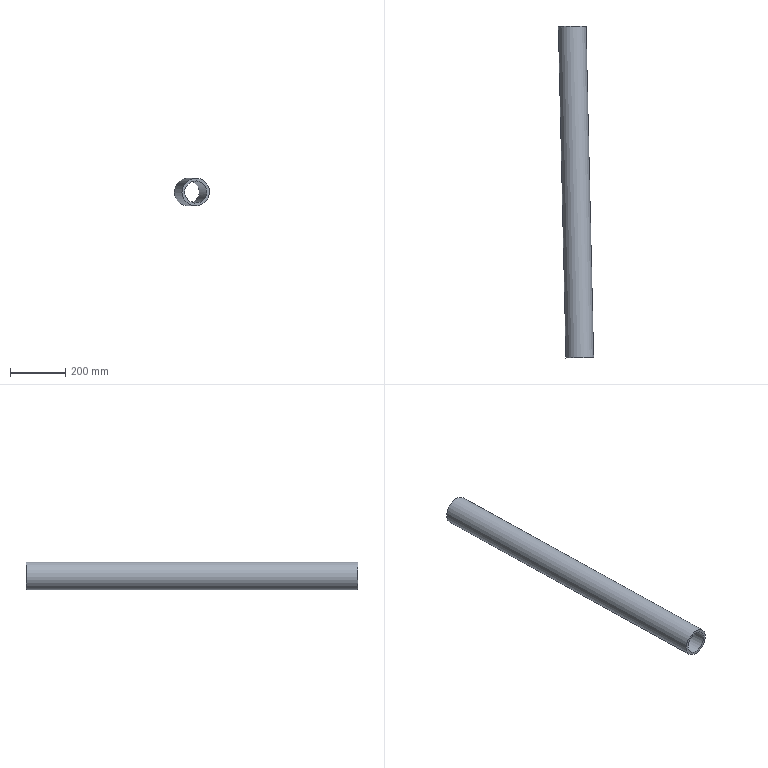Component | NX | 5 | 1 solid | 4 faces | box 127.4 x 1201.97 x 100 mm | volume 3392920 mm3 | plane 2 | cylinder 2 | commonest cylinder face diameters 100 x1 80 x1
STEP:
#1=CARTESIAN_POINT('',(0.,0.,0.));
#2=DIRECTION('',(0.,0.,1.));
#3=DIRECTION('',(1.,0.,0.));
#4=AXIS2_PLACEMENT_3D('',#1,#2,#3);
#5=CARTESIAN_POINT('',(-401.993,544.191,132.036));
#6=VERTEX_POINT('',#5);
#7=CARTESIAN_POINT('',(-421.336,543.749,185.193));
#8=VERTEX_POINT('',#7);
#9=CARTESIAN_POINT('',(-385.093,544.578,168.288));
#10=DIRECTION('',(0.02285,-0.9997,0.));
#11=DIRECTION('',(-0.4225,-0.009659,-0.9063));
#12=AXIS2_PLACEMENT_3D('',#9,#10,#11);
#13=CIRCLE('',#12,40.);
#14=CARTESIAN_POINT('',(-385.093,544.578,168.288));
#15=DIRECTION('',(-0.02285,0.9997,0.));
#16=DIRECTION('',(-0.4225,-0.009659,-0.9063));
#17=AXIS2_PLACEMENT_3D('',#14,#15,#16);
#18=PLANE('',#17);
#19=CARTESIAN_POINT('',(40.,0.));
#20=CARTESIAN_POINT('',(40.,-69.282));
#21=CARTESIAN_POINT('',(-20.,-34.641));
#22=CARTESIAN_POINT('',(-80.,-0.));
#23=CARTESIAN_POINT('',(-20.,34.641));
#24=CARTESIAN_POINT('',(40.,69.282));
#25=CARTESIAN_POINT('',(40.,0.));
#26=(BOUNDED_CURVE()B_SPLINE_CURVE(2,(#19,#20,#21,#22,#23,#24,#25),.UNSPECIFIED.,.T.,.F.)B_SPLINE_CURVE_WITH_KNOTS((1,2,2,2,2,1),(-2.094,0.,2.094,4.189,6.283,8.378),.UNSPECIFIED.)CURVE()GEOMETRIC_REPRESENTATION_ITEM()RATIONAL_B_SPLINE_CURVE((1.,0.5,1.,0.5,1.,0.5,1.))REPRESENTATION_ITEM(''));
#27=(GEOMETRIC_REPRESENTATION_CONTEXT(2)PARAMETRIC_REPRESENTATION_CONTEXT()REPRESENTATION_CONTEXT('',''));
#28=DEFINITIONAL_REPRESENTATION('',(#26),#27);
#29=PCURVE('',#18,#28);
#30=CARTESIAN_POINT('',(-357.668,-655.109,168.288));
#31=DIRECTION('',(-0.02285,0.9997,0.));
#32=DIRECTION('',(-0.9061,-0.02071,0.4226));
#33=AXIS2_PLACEMENT_3D('',#30,#31,#32);
#34=CYLINDRICAL_SURFACE('',#33,40.);
#35=CARTESIAN_POINT('',(4.712,1200.));
#36=DIRECTION('',(-1.,0.));
#37=VECTOR('',#36,1.);
#38=LINE('',#35,#37);
#39=(GEOMETRIC_REPRESENTATION_CONTEXT(2)PARAMETRIC_REPRESENTATION_CONTEXT()REPRESENTATION_CONTEXT('',''));
#40=DEFINITIONAL_REPRESENTATION('',(#38),#39);
#41=PCURVE('',#34,#40);
#42=SURFACE_CURVE('',#13,(#29,#41),.PCURVE_S1.);
#43=EDGE_CURVE('',#6,#8,#42,.T.);
#44=ORIENTED_EDGE('',*,*,#43,.T.);
#45=CARTESIAN_POINT('',(-385.093,544.578,168.288));
#46=DIRECTION('',(0.02285,-0.9997,0.));
#47=DIRECTION('',(-0.4225,-0.009659,-0.9063));
#48=AXIS2_PLACEMENT_3D('',#45,#46,#47);
#49=CIRCLE('',#48,40.);
#50=CARTESIAN_POINT('',(40.,0.));
#51=CARTESIAN_POINT('',(40.,-69.282));
#52=CARTESIAN_POINT('',(-20.,-34.641));
#53=CARTESIAN_POINT('',(-80.,-0.));
#54=CARTESIAN_POINT('',(-20.,34.641));
#55=CARTESIAN_POINT('',(40.,69.282));
#56=CARTESIAN_POINT('',(40.,0.));
#57=(BOUNDED_CURVE()B_SPLINE_CURVE(2,(#50,#51,#52,#53,#54,#55,#56),.UNSPECIFIED.,.T.,.F.)B_SPLINE_CURVE_WITH_KNOTS((1,2,2,2,2,1),(-2.094,0.,2.094,4.189,6.283,8.378),.UNSPECIFIED.)CURVE()GEOMETRIC_REPRESENTATION_ITEM()RATIONAL_B_SPLINE_CURVE((1.,0.5,1.,0.5,1.,0.5,1.))REPRESENTATION_ITEM(''));
#58=(GEOMETRIC_REPRESENTATION_CONTEXT(2)PARAMETRIC_REPRESENTATION_CONTEXT()REPRESENTATION_CONTEXT('',''));
#59=DEFINITIONAL_REPRESENTATION('',(#57),#58);
#60=PCURVE('',#18,#59);
#61=CARTESIAN_POINT('',(10.996,1200.));
#62=DIRECTION('',(-1.,0.));
#63=VECTOR('',#62,1.);
#64=LINE('',#61,#63);
#65=(GEOMETRIC_REPRESENTATION_CONTEXT(2)PARAMETRIC_REPRESENTATION_CONTEXT()REPRESENTATION_CONTEXT('',''));
#66=DEFINITIONAL_REPRESENTATION('',(#64),#65);
#67=PCURVE('',#34,#66);
#68=SURFACE_CURVE('',#49,(#60,#67),.PCURVE_S1.);
#69=EDGE_CURVE('',#8,#6,#68,.T.);
#70=ORIENTED_EDGE('',*,*,#69,.T.);
#71=EDGE_LOOP('',(#44,#70));
#72=FACE_BOUND('',#71,.T.);
#73=CARTESIAN_POINT('',(-430.396,543.542,189.419));
#74=VERTEX_POINT('',#73);
#75=CARTESIAN_POINT('',(-385.093,544.578,168.288));
#76=DIRECTION('',(0.02285,-0.9997,-0.));
#77=DIRECTION('',(-0.9061,-0.02071,0.4226));
#78=AXIS2_PLACEMENT_3D('',#75,#76,#77);
#79=CIRCLE('',#78,50.);
#80=CARTESIAN_POINT('',(0.,50.));
#81=CARTESIAN_POINT('',(86.603,50.));
#82=CARTESIAN_POINT('',(43.301,-25.));
#83=CARTESIAN_POINT('',(-0.,-100.));
#84=CARTESIAN_POINT('',(-43.301,-25.));
#85=CARTESIAN_POINT('',(-86.603,50.));
#86=CARTESIAN_POINT('',(0.,50.));
#87=(BOUNDED_CURVE()B_SPLINE_CURVE(2,(#80,#81,#82,#83,#84,#85,#86),.UNSPECIFIED.,.T.,.F.)B_SPLINE_CURVE_WITH_KNOTS((1,2,2,2,2,1),(-2.094,0.,2.094,4.189,6.283,8.378),.UNSPECIFIED.)CURVE()GEOMETRIC_REPRESENTATION_ITEM()RATIONAL_B_SPLINE_CURVE((1.,0.5,1.,0.5,1.,0.5,1.))REPRESENTATION_ITEM(''));
#88=(GEOMETRIC_REPRESENTATION_CONTEXT(2)PARAMETRIC_REPRESENTATION_CONTEXT()REPRESENTATION_CONTEXT('',''));
#89=DEFINITIONAL_REPRESENTATION('',(#87),#88);
#90=PCURVE('',#18,#89);
#91=CARTESIAN_POINT('',(-357.668,-655.109,168.288));
#92=DIRECTION('',(-0.02285,0.9997,0.));
#93=DIRECTION('',(-0.9061,-0.02071,0.4226));
#94=AXIS2_PLACEMENT_3D('',#91,#92,#93);
#95=CYLINDRICAL_SURFACE('',#94,50.);
#96=CARTESIAN_POINT('',(6.283,1200.));
#97=DIRECTION('',(-1.,0.));
#98=VECTOR('',#97,1.);
#99=LINE('',#96,#98);
#100=(GEOMETRIC_REPRESENTATION_CONTEXT(2)PARAMETRIC_REPRESENTATION_CONTEXT()REPRESENTATION_CONTEXT('',''));
#101=DEFINITIONAL_REPRESENTATION('',(#99),#100);
#102=PCURVE('',#95,#101);
#103=SURFACE_CURVE('',#79,(#90,#102),.PCURVE_S1.);
#104=EDGE_CURVE('',#74,#74,#103,.T.);
#105=ORIENTED_EDGE('',*,*,#104,.F.);
#106=EDGE_LOOP('',(#105));
#107=FACE_BOUND('',#106,.T.);
#108=ADVANCED_FACE('',(#72,#107),#18,.T.);
#109=CARTESIAN_POINT('',(-393.911,-655.937,185.193));
#110=VERTEX_POINT('',#109);
#111=CARTESIAN_POINT('',(-357.668,-655.109,168.288));
#112=DIRECTION('',(-0.02285,0.9997,0.));
#113=DIRECTION('',(-0.9061,-0.02071,0.4226));
#114=AXIS2_PLACEMENT_3D('',#111,#112,#113);
#115=CIRCLE('',#114,40.);
#116=CARTESIAN_POINT('',(-357.668,-655.109,168.288));
#117=DIRECTION('',(0.02285,-0.9997,0.));
#118=DIRECTION('',(0.4225,0.009659,0.9063));
#119=AXIS2_PLACEMENT_3D('',#116,#117,#118);
#120=PLANE('',#119);
#121=CARTESIAN_POINT('',(0.,40.));
#122=CARTESIAN_POINT('',(69.282,40.));
#123=CARTESIAN_POINT('',(34.641,-20.));
#124=CARTESIAN_POINT('',(-0.,-80.));
#125=CARTESIAN_POINT('',(-34.641,-20.));
#126=CARTESIAN_POINT('',(-69.282,40.));
#127=CARTESIAN_POINT('',(0.,40.));
#128=(BOUNDED_CURVE()B_SPLINE_CURVE(2,(#121,#122,#123,#124,#125,#126,#127),.UNSPECIFIED.,.T.,.F.)B_SPLINE_CURVE_WITH_KNOTS((1,2,2,2,2,1),(-2.094,0.,2.094,4.189,6.283,8.378),.UNSPECIFIED.)CURVE()GEOMETRIC_REPRESENTATION_ITEM()RATIONAL_B_SPLINE_CURVE((1.,0.5,1.,0.5,1.,0.5,1.))REPRESENTATION_ITEM(''));
#129=(GEOMETRIC_REPRESENTATION_CONTEXT(2)PARAMETRIC_REPRESENTATION_CONTEXT()REPRESENTATION_CONTEXT('',''));
#130=DEFINITIONAL_REPRESENTATION('',(#128),#129);
#131=PCURVE('',#120,#130);
#132=CARTESIAN_POINT('',(0.,0.));
#133=DIRECTION('',(1.,0.));
#134=VECTOR('',#133,1.);
#135=LINE('',#132,#134);
#136=(GEOMETRIC_REPRESENTATION_CONTEXT(2)PARAMETRIC_REPRESENTATION_CONTEXT()REPRESENTATION_CONTEXT('',''));
#137=DEFINITIONAL_REPRESENTATION('',(#135),#136);
#138=PCURVE('',#34,#137);
#139=SURFACE_CURVE('',#115,(#131,#138),.PCURVE_S1.);
#140=EDGE_CURVE('',#110,#110,#139,.T.);
#141=ORIENTED_EDGE('',*,*,#140,.T.);
#142=EDGE_LOOP('',(#141));
#143=FACE_BOUND('',#142,.T.);
#144=CARTESIAN_POINT('',(-402.971,-656.144,189.419));
#145=VERTEX_POINT('',#144);
#146=CARTESIAN_POINT('',(-357.668,-655.109,168.288));
#147=DIRECTION('',(-0.02285,0.9997,0.));
#148=DIRECTION('',(-0.9061,-0.02071,0.4226));
#149=AXIS2_PLACEMENT_3D('',#146,#147,#148);
#150=CIRCLE('',#149,50.);
#151=CARTESIAN_POINT('',(-0.,50.));
#152=CARTESIAN_POINT('',(86.603,50.));
#153=CARTESIAN_POINT('',(43.301,-25.));
#154=CARTESIAN_POINT('',(0.,-100.));
#155=CARTESIAN_POINT('',(-43.301,-25.));
#156=CARTESIAN_POINT('',(-86.603,50.));
#157=CARTESIAN_POINT('',(-0.,50.));
#158=(BOUNDED_CURVE()B_SPLINE_CURVE(2,(#151,#152,#153,#154,#155,#156,#157),.UNSPECIFIED.,.T.,.F.)B_SPLINE_CURVE_WITH_KNOTS((1,2,2,2,2,1),(-2.094,0.,2.094,4.189,6.283,8.378),.UNSPECIFIED.)CURVE()GEOMETRIC_REPRESENTATION_ITEM()RATIONAL_B_SPLINE_CURVE((1.,0.5,1.,0.5,1.,0.5,1.))REPRESENTATION_ITEM(''));
#159=(GEOMETRIC_REPRESENTATION_CONTEXT(2)PARAMETRIC_REPRESENTATION_CONTEXT()REPRESENTATION_CONTEXT('',''));
#160=DEFINITIONAL_REPRESENTATION('',(#158),#159);
#161=PCURVE('',#120,#160);
#162=CARTESIAN_POINT('',(0.,0.));
#163=DIRECTION('',(1.,0.));
#164=VECTOR('',#163,1.);
#165=LINE('',#162,#164);
#166=(GEOMETRIC_REPRESENTATION_CONTEXT(2)PARAMETRIC_REPRESENTATION_CONTEXT()REPRESENTATION_CONTEXT('',''));
#167=DEFINITIONAL_REPRESENTATION('',(#165),#166);
#168=PCURVE('',#95,#167);
#169=SURFACE_CURVE('',#150,(#161,#168),.PCURVE_S1.);
#170=EDGE_CURVE('',#145,#145,#169,.T.);
#171=ORIENTED_EDGE('',*,*,#170,.F.);
#172=EDGE_LOOP('',(#171));
#173=FACE_BOUND('',#172,.T.);
#174=ADVANCED_FACE('',(#143,#173),#120,.T.);
#175=ORIENTED_EDGE('',*,*,#104,.T.);
#176=CARTESIAN_POINT('',(-402.971,-656.144,189.419));
#177=CARTESIAN_POINT('',(-430.396,543.542,189.419));
#178=B_SPLINE_CURVE_WITH_KNOTS('',1,(#176,#177),.UNSPECIFIED.,.F.,.F.,(2,2),(0.,1200.),.PIECEWISE_BEZIER_KNOTS.);
#179=CARTESIAN_POINT('',(0.,0.));
#180=DIRECTION('',(0.,1.));
#181=VECTOR('',#180,1.);
#182=LINE('',#179,#181);
#183=(GEOMETRIC_REPRESENTATION_CONTEXT(2)PARAMETRIC_REPRESENTATION_CONTEXT()REPRESENTATION_CONTEXT('',''));
#184=DEFINITIONAL_REPRESENTATION('',(#182),#183);
#185=PCURVE('',#95,#184);
#186=CARTESIAN_POINT('',(6.283,0.));
#187=DIRECTION('',(0.,1.));
#188=VECTOR('',#187,1.);
#189=LINE('',#186,#188);
#190=(GEOMETRIC_REPRESENTATION_CONTEXT(2)PARAMETRIC_REPRESENTATION_CONTEXT()REPRESENTATION_CONTEXT('',''));
#191=DEFINITIONAL_REPRESENTATION('',(#189),#190);
#192=PCURVE('',#95,#191);
#193=SEAM_CURVE('',#178,(#185,#192),.PCURVE_S1.);
#194=EDGE_CURVE('',#145,#74,#193,.T.);
#195=ORIENTED_EDGE('',*,*,#194,.F.);
#196=ORIENTED_EDGE('',*,*,#170,.T.);
#197=ORIENTED_EDGE('',*,*,#194,.T.);
#198=EDGE_LOOP('',(#175,#195,#196,#197));
#199=FACE_BOUND('',#198,.T.);
#200=ADVANCED_FACE('',(#199),#95,.T.);
#201=ORIENTED_EDGE('',*,*,#43,.T.);
#202=CARTESIAN_POINT('',(-393.911,-655.937,185.193));
#203=CARTESIAN_POINT('',(-421.336,543.749,185.193));
#204=B_SPLINE_CURVE_WITH_KNOTS('',1,(#202,#203),.UNSPECIFIED.,.F.,.F.,(2,2),(0.,1200.),.PIECEWISE_BEZIER_KNOTS.);
#205=CARTESIAN_POINT('',(0.,0.));
#206=DIRECTION('',(0.,1.));
#207=VECTOR('',#206,1.);
#208=LINE('',#205,#207);
#209=(GEOMETRIC_REPRESENTATION_CONTEXT(2)PARAMETRIC_REPRESENTATION_CONTEXT()REPRESENTATION_CONTEXT('',''));
#210=DEFINITIONAL_REPRESENTATION('',(#208),#209);
#211=PCURVE('',#34,#210);
#212=CARTESIAN_POINT('',(6.283,0.));
#213=DIRECTION('',(0.,1.));
#214=VECTOR('',#213,1.);
#215=LINE('',#212,#214);
#216=(GEOMETRIC_REPRESENTATION_CONTEXT(2)PARAMETRIC_REPRESENTATION_CONTEXT()REPRESENTATION_CONTEXT('',''));
#217=DEFINITIONAL_REPRESENTATION('',(#215),#216);
#218=PCURVE('',#34,#217);
#219=SEAM_CURVE('',#204,(#211,#218),.PCURVE_S1.);
#220=EDGE_CURVE('',#110,#8,#219,.T.);
#221=ORIENTED_EDGE('',*,*,#220,.F.);
#222=ORIENTED_EDGE('',*,*,#140,.T.);
#223=ORIENTED_EDGE('',*,*,#220,.T.);
#224=ORIENTED_EDGE('',*,*,#69,.T.);
#225=EDGE_LOOP('',(#201,#221,#222,#223,#224));
#226=FACE_BOUND('',#225,.F.);
#227=ADVANCED_FACE('',(#226),#34,.F.);
#228=CLOSED_SHELL('',(#108,#174,#200,#227));
#229=MANIFOLD_SOLID_BREP('',#228);
#230=(LENGTH_UNIT()NAMED_UNIT(*)SI_UNIT(.MILLI.,.METRE.));
#231=UNCERTAINTY_MEASURE_WITH_UNIT(LENGTH_MEASURE(0.000005),#230,'','');
#232=(NAMED_UNIT(*)PLANE_ANGLE_UNIT()SI_UNIT($,.RADIAN.));
#233=(NAMED_UNIT(*)SI_UNIT($,.STERADIAN.)SOLID_ANGLE_UNIT());
#234=(GEOMETRIC_REPRESENTATION_CONTEXT(3)GLOBAL_UNCERTAINTY_ASSIGNED_CONTEXT((#231))GLOBAL_UNIT_ASSIGNED_CONTEXT((#230,#232,#233))REPRESENTATION_CONTEXT('',''));
#235=ADVANCED_BREP_SHAPE_REPRESENTATION('',(#4,#229),#234);